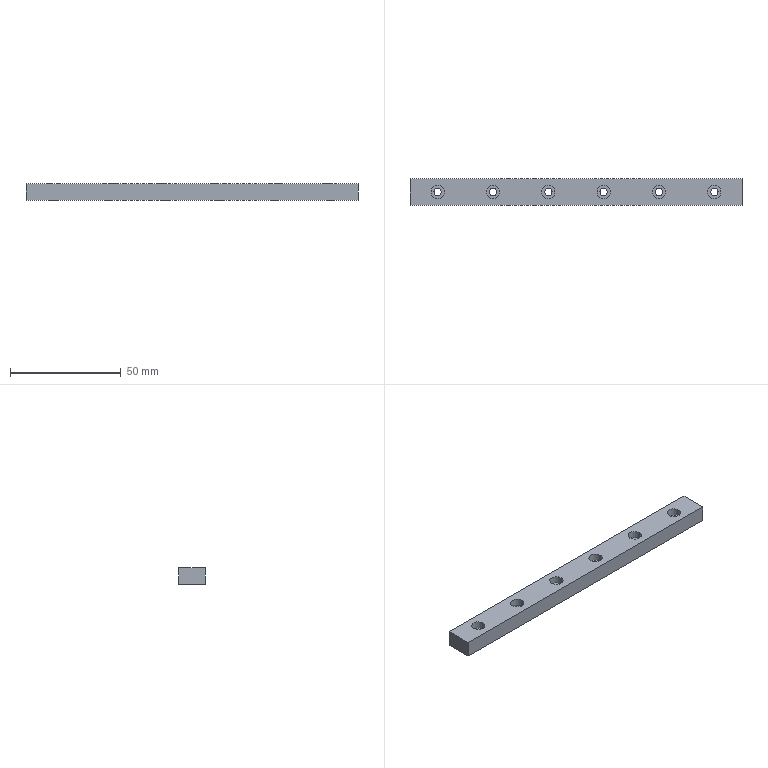Component | SolidWorks | TM12NNA-1-150-NA-Z0-1_TM12NN-150-1 | 1 solid | 36 faces | box 150 x 12 x 7.5 mm | volume 12700 mm3 | cylinder 24 | plane 12 | commonest cylinder face diameters 3.4 x12 6 x12 | material 45
build123d program:
from build123d import *

# Parameters (mm, degrees)
SKETCH1_W                                          = 12
SKETCH1_H                                          = 7.5
BOSS_EXTRUDE1_DEPTH                                = 75
HOLE_SIZE_ACCORDING_TO_TYPE_OF_HEXAGON_D           = 3.4
HOLE_SIZE_ACCORDING_TO_TYPE_OF_HEXAGON_CBORE_D     = 6
HOLE_SIZE_ACCORDING_TO_TYPE_OF_HEXAGON_CBORE_DEPTH = 3.4
LPATTERN1_COUNT                                    = 6
LPATTERN1_PITCH                                    = 25


with BuildPart() as part:
    # Sketch1 → Boss-Extrude1 (new, symmetric)
    with BuildSketch(Plane.XY):
        Rectangle(SKETCH1_W, SKETCH1_H)
    extrude(amount=BOSS_EXTRUDE1_DEPTH, both=True)

    # Hole Size _According to_ Type of Hexagon (through all)
    with Locations(Plane(origin=(0, 3.75, 0), x_dir=(1, 0, 0), z_dir=(0, 1, 0))):
        with Locations((0, -62.5)):
            hole_size_according_to_type_of_hexagon = CounterBoreHole(HOLE_SIZE_ACCORDING_TO_TYPE_OF_HEXAGON_D / 2, HOLE_SIZE_ACCORDING_TO_TYPE_OF_HEXAGON_CBORE_D / 2, HOLE_SIZE_ACCORDING_TO_TYPE_OF_HEXAGON_CBORE_DEPTH)

    # LPattern1: Hole Size _According to_ Type of Hexagon ×6
    with Locations(*[(0, 0, -i * LPATTERN1_PITCH) for i in range(1, LPATTERN1_COUNT)]):
        add(hole_size_according_to_type_of_hexagon, mode=Mode.SUBTRACT)


solid = part.part

# Placed as in the assembly
solid = solid.moved(Location((205, 24, -71.25), (90, -90, 0)))
STEP:
#1=COLOUR_RGB('',0.7922,0.8196,0.9333);
#2=FILL_AREA_STYLE_COLOUR('',#1);
#3=FILL_AREA_STYLE('',(#2));
#4=SURFACE_STYLE_FILL_AREA(#3);
#5=SURFACE_SIDE_STYLE('',(#4));
#6=SURFACE_STYLE_USAGE(.BOTH.,#5);
#7=PRESENTATION_STYLE_ASSIGNMENT((#6));
#8=CARTESIAN_POINT('',(5.543,0.9449,-2.953));
#9=VERTEX_POINT('',#8);
#10=CARTESIAN_POINT('',(5.677,0.9449,-2.953));
#11=VERTEX_POINT('',#10);
#12=CARTESIAN_POINT('',(5.61,0.9449,-2.953));
#13=DIRECTION('',(0.,0.,1.));
#14=DIRECTION('',(1.,0.,0.));
#15=AXIS2_PLACEMENT_3D('',#12,#13,#14);
#16=CIRCLE('',#15,0.06693);
#17=EDGE_CURVE('',#9,#11,#16,.T.);
#18=ORIENTED_EDGE('',*,*,#17,.F.);
#19=CARTESIAN_POINT('',(5.543,0.9449,-2.791));
#20=VERTEX_POINT('',#19);
#21=CARTESIAN_POINT('',(5.543,0.9449,-2.657));
#22=DIRECTION('',(0.,0.,1.));
#23=VECTOR('',#22,39.37);
#24=LINE('',#21,#23);
#25=EDGE_CURVE('',#9,#20,#24,.T.);
#26=ORIENTED_EDGE('',*,*,#25,.T.);
#27=CARTESIAN_POINT('',(5.677,0.9449,-2.791));
#28=VERTEX_POINT('',#27);
#29=CARTESIAN_POINT('',(5.61,0.9449,-2.791));
#30=DIRECTION('',(0.,0.,1.));
#31=DIRECTION('',(1.,0.,0.));
#32=AXIS2_PLACEMENT_3D('',#29,#30,#31);
#33=CIRCLE('',#32,0.06693);
#34=EDGE_CURVE('',#20,#28,#33,.T.);
#35=ORIENTED_EDGE('',*,*,#34,.T.);
#36=CARTESIAN_POINT('',(5.677,0.9449,-2.657));
#37=DIRECTION('',(0.,0.,1.));
#38=VECTOR('',#37,39.37);
#39=LINE('',#36,#38);
#40=EDGE_CURVE('',#11,#28,#39,.T.);
#41=ORIENTED_EDGE('',*,*,#40,.F.);
#42=EDGE_LOOP('',(#18,#26,#35,#41));
#43=FACE_OUTER_BOUND('',#42,.T.);
#44=CARTESIAN_POINT('',(5.61,0.9449,-2.657));
#45=DIRECTION('',(0.,0.,1.));
#46=DIRECTION('',(1.,0.,0.));
#47=AXIS2_PLACEMENT_3D('',#44,#45,#46);
#48=CYLINDRICAL_SURFACE('',#47,0.06693);
#49=ADVANCED_FACE('',(#43),#48,.F.);
#50=CARTESIAN_POINT('',(5.492,0.9449,-2.791));
#51=VERTEX_POINT('',#50);
#52=CARTESIAN_POINT('',(5.728,0.9449,-2.791));
#53=VERTEX_POINT('',#52);
#54=CARTESIAN_POINT('',(5.61,0.9449,-2.791));
#55=DIRECTION('',(0.,0.,1.));
#56=DIRECTION('',(1.,0.,0.));
#57=AXIS2_PLACEMENT_3D('',#54,#55,#56);
#58=CIRCLE('',#57,0.1181);
#59=EDGE_CURVE('',#51,#53,#58,.T.);
#60=ORIENTED_EDGE('',*,*,#59,.F.);
#61=CARTESIAN_POINT('',(5.492,0.9449,-2.657));
#62=VERTEX_POINT('',#61);
#63=CARTESIAN_POINT('',(5.492,0.9449,-2.657));
#64=DIRECTION('',(0.,0.,1.));
#65=VECTOR('',#64,39.37);
#66=LINE('',#63,#65);
#67=EDGE_CURVE('',#51,#62,#66,.T.);
#68=ORIENTED_EDGE('',*,*,#67,.T.);
#69=CARTESIAN_POINT('',(5.728,0.9449,-2.657));
#70=VERTEX_POINT('',#69);
#71=CARTESIAN_POINT('',(5.61,0.9449,-2.657));
#72=DIRECTION('',(0.,0.,1.));
#73=DIRECTION('',(1.,0.,0.));
#74=AXIS2_PLACEMENT_3D('',#71,#72,#73);
#75=CIRCLE('',#74,0.1181);
#76=EDGE_CURVE('',#62,#70,#75,.T.);
#77=ORIENTED_EDGE('',*,*,#76,.T.);
#78=CARTESIAN_POINT('',(5.728,0.9449,-2.657));
#79=DIRECTION('',(0.,0.,1.));
#80=VECTOR('',#79,39.37);
#81=LINE('',#78,#80);
#82=EDGE_CURVE('',#53,#70,#81,.T.);
#83=ORIENTED_EDGE('',*,*,#82,.F.);
#84=EDGE_LOOP('',(#60,#68,#77,#83));
#85=FACE_OUTER_BOUND('',#84,.T.);
#86=CARTESIAN_POINT('',(5.61,0.9449,-2.657));
#87=DIRECTION('',(0.,0.,1.));
#88=DIRECTION('',(1.,0.,0.));
#89=AXIS2_PLACEMENT_3D('',#86,#87,#88);
#90=CYLINDRICAL_SURFACE('',#89,0.1181);
#91=ADVANCED_FACE('',(#85),#90,.F.);
#92=CARTESIAN_POINT('',(6.528,0.9449,-2.953));
#93=VERTEX_POINT('',#92);
#94=CARTESIAN_POINT('',(6.661,0.9449,-2.953));
#95=VERTEX_POINT('',#94);
#96=CARTESIAN_POINT('',(6.594,0.9449,-2.953));
#97=DIRECTION('',(0.,0.,1.));
#98=DIRECTION('',(1.,0.,0.));
#99=AXIS2_PLACEMENT_3D('',#96,#97,#98);
#100=CIRCLE('',#99,0.06693);
#101=EDGE_CURVE('',#93,#95,#100,.T.);
#102=ORIENTED_EDGE('',*,*,#101,.F.);
#103=CARTESIAN_POINT('',(6.528,0.9449,-2.791));
#104=VERTEX_POINT('',#103);
#105=CARTESIAN_POINT('',(6.528,0.9449,-2.657));
#106=DIRECTION('',(0.,0.,1.));
#107=VECTOR('',#106,39.37);
#108=LINE('',#105,#107);
#109=EDGE_CURVE('',#93,#104,#108,.T.);
#110=ORIENTED_EDGE('',*,*,#109,.T.);
#111=CARTESIAN_POINT('',(6.661,0.9449,-2.791));
#112=VERTEX_POINT('',#111);
#113=CARTESIAN_POINT('',(6.594,0.9449,-2.791));
#114=DIRECTION('',(0.,0.,1.));
#115=DIRECTION('',(1.,0.,0.));
#116=AXIS2_PLACEMENT_3D('',#113,#114,#115);
#117=CIRCLE('',#116,0.06693);
#118=EDGE_CURVE('',#104,#112,#117,.T.);
#119=ORIENTED_EDGE('',*,*,#118,.T.);
#120=CARTESIAN_POINT('',(6.661,0.9449,-2.657));
#121=DIRECTION('',(0.,0.,1.));
#122=VECTOR('',#121,39.37);
#123=LINE('',#120,#122);
#124=EDGE_CURVE('',#95,#112,#123,.T.);
#125=ORIENTED_EDGE('',*,*,#124,.F.);
#126=EDGE_LOOP('',(#102,#110,#119,#125));
#127=FACE_OUTER_BOUND('',#126,.T.);
#128=CARTESIAN_POINT('',(6.594,0.9449,-2.657));
#129=DIRECTION('',(0.,0.,1.));
#130=DIRECTION('',(1.,0.,0.));
#131=AXIS2_PLACEMENT_3D('',#128,#129,#130);
#132=CYLINDRICAL_SURFACE('',#131,0.06693);
#133=ADVANCED_FACE('',(#127),#132,.F.);
#134=CARTESIAN_POINT('',(6.476,0.9449,-2.791));
#135=VERTEX_POINT('',#134);
#136=CARTESIAN_POINT('',(6.713,0.9449,-2.791));
#137=VERTEX_POINT('',#136);
#138=CARTESIAN_POINT('',(6.594,0.9449,-2.791));
#139=DIRECTION('',(0.,0.,1.));
#140=DIRECTION('',(1.,0.,0.));
#141=AXIS2_PLACEMENT_3D('',#138,#139,#140);
#142=CIRCLE('',#141,0.1181);
#143=EDGE_CURVE('',#135,#137,#142,.T.);
#144=ORIENTED_EDGE('',*,*,#143,.F.);
#145=CARTESIAN_POINT('',(6.476,0.9449,-2.657));
#146=VERTEX_POINT('',#145);
#147=CARTESIAN_POINT('',(6.476,0.9449,-2.657));
#148=DIRECTION('',(0.,0.,1.));
#149=VECTOR('',#148,39.37);
#150=LINE('',#147,#149);
#151=EDGE_CURVE('',#135,#146,#150,.T.);
#152=ORIENTED_EDGE('',*,*,#151,.T.);
#153=CARTESIAN_POINT('',(6.713,0.9449,-2.657));
#154=VERTEX_POINT('',#153);
#155=CARTESIAN_POINT('',(6.594,0.9449,-2.657));
#156=DIRECTION('',(0.,0.,1.));
#157=DIRECTION('',(1.,0.,0.));
#158=AXIS2_PLACEMENT_3D('',#155,#156,#157);
#159=CIRCLE('',#158,0.1181);
#160=EDGE_CURVE('',#146,#154,#159,.T.);
#161=ORIENTED_EDGE('',*,*,#160,.T.);
#162=CARTESIAN_POINT('',(6.713,0.9449,-2.657));
#163=DIRECTION('',(0.,0.,1.));
#164=VECTOR('',#163,39.37);
#165=LINE('',#162,#164);
#166=EDGE_CURVE('',#137,#154,#165,.T.);
#167=ORIENTED_EDGE('',*,*,#166,.F.);
#168=EDGE_LOOP('',(#144,#152,#161,#167));
#169=FACE_OUTER_BOUND('',#168,.T.);
#170=CARTESIAN_POINT('',(6.594,0.9449,-2.657));
#171=DIRECTION('',(0.,0.,1.));
#172=DIRECTION('',(1.,0.,0.));
#173=AXIS2_PLACEMENT_3D('',#170,#171,#172);
#174=CYLINDRICAL_SURFACE('',#173,0.1181);
#175=ADVANCED_FACE('',(#169),#174,.F.);
#176=CARTESIAN_POINT('',(7.512,0.9449,-2.953));
#177=VERTEX_POINT('',#176);
#178=CARTESIAN_POINT('',(7.646,0.9449,-2.953));
#179=VERTEX_POINT('',#178);
#180=CARTESIAN_POINT('',(7.579,0.9449,-2.953));
#181=DIRECTION('',(0.,0.,1.));
#182=DIRECTION('',(1.,0.,0.));
#183=AXIS2_PLACEMENT_3D('',#180,#181,#182);
#184=CIRCLE('',#183,0.06693);
#185=EDGE_CURVE('',#177,#179,#184,.T.);
#186=ORIENTED_EDGE('',*,*,#185,.F.);
#187=CARTESIAN_POINT('',(7.512,0.9449,-2.791));
#188=VERTEX_POINT('',#187);
#189=CARTESIAN_POINT('',(7.512,0.9449,-2.657));
#190=DIRECTION('',(0.,0.,1.));
#191=VECTOR('',#190,39.37);
#192=LINE('',#189,#191);
#193=EDGE_CURVE('',#177,#188,#192,.T.);
#194=ORIENTED_EDGE('',*,*,#193,.T.);
#195=CARTESIAN_POINT('',(7.646,0.9449,-2.791));
#196=VERTEX_POINT('',#195);
#197=CARTESIAN_POINT('',(7.579,0.9449,-2.791));
#198=DIRECTION('',(0.,0.,1.));
#199=DIRECTION('',(1.,0.,0.));
#200=AXIS2_PLACEMENT_3D('',#197,#198,#199);
#201=CIRCLE('',#200,0.06693);
#202=EDGE_CURVE('',#188,#196,#201,.T.);
#203=ORIENTED_EDGE('',*,*,#202,.T.);
#204=CARTESIAN_POINT('',(7.646,0.9449,-2.657));
#205=DIRECTION('',(0.,0.,1.));
#206=VECTOR('',#205,39.37);
#207=LINE('',#204,#206);
#208=EDGE_CURVE('',#179,#196,#207,.T.);
#209=ORIENTED_EDGE('',*,*,#208,.F.);
#210=EDGE_LOOP('',(#186,#194,#203,#209));
#211=FACE_OUTER_BOUND('',#210,.T.);
#212=CARTESIAN_POINT('',(7.579,0.9449,-2.657));
#213=DIRECTION('',(0.,0.,1.));
#214=DIRECTION('',(1.,0.,0.));
#215=AXIS2_PLACEMENT_3D('',#212,#213,#214);
#216=CYLINDRICAL_SURFACE('',#215,0.06693);
#217=ADVANCED_FACE('',(#211),#216,.F.);
#218=CARTESIAN_POINT('',(7.461,0.9449,-2.791));
#219=VERTEX_POINT('',#218);
#220=CARTESIAN_POINT('',(7.697,0.9449,-2.791));
#221=VERTEX_POINT('',#220);
#222=CARTESIAN_POINT('',(7.579,0.9449,-2.791));
#223=DIRECTION('',(0.,0.,1.));
#224=DIRECTION('',(1.,0.,0.));
#225=AXIS2_PLACEMENT_3D('',#222,#223,#224);
#226=CIRCLE('',#225,0.1181);
#227=EDGE_CURVE('',#219,#221,#226,.T.);
#228=ORIENTED_EDGE('',*,*,#227,.F.);
#229=CARTESIAN_POINT('',(7.461,0.9449,-2.657));
#230=VERTEX_POINT('',#229);
#231=CARTESIAN_POINT('',(7.461,0.9449,-2.657));
#232=DIRECTION('',(0.,0.,1.));
#233=VECTOR('',#232,39.37);
#234=LINE('',#231,#233);
#235=EDGE_CURVE('',#219,#230,#234,.T.);
#236=ORIENTED_EDGE('',*,*,#235,.T.);
#237=CARTESIAN_POINT('',(7.697,0.9449,-2.657));
#238=VERTEX_POINT('',#237);
#239=CARTESIAN_POINT('',(7.579,0.9449,-2.657));
#240=DIRECTION('',(0.,0.,1.));
#241=DIRECTION('',(1.,0.,0.));
#242=AXIS2_PLACEMENT_3D('',#239,#240,#241);
#243=CIRCLE('',#242,0.1181);
#244=EDGE_CURVE('',#230,#238,#243,.T.);
#245=ORIENTED_EDGE('',*,*,#244,.T.);
#246=CARTESIAN_POINT('',(7.697,0.9449,-2.657));
#247=DIRECTION('',(0.,0.,1.));
#248=VECTOR('',#247,39.37);
#249=LINE('',#246,#248);
#250=EDGE_CURVE('',#221,#238,#249,.T.);
#251=ORIENTED_EDGE('',*,*,#250,.F.);
#252=EDGE_LOOP('',(#228,#236,#245,#251));
#253=FACE_OUTER_BOUND('',#252,.T.);
#254=CARTESIAN_POINT('',(7.579,0.9449,-2.657));
#255=DIRECTION('',(0.,0.,1.));
#256=DIRECTION('',(1.,0.,0.));
#257=AXIS2_PLACEMENT_3D('',#254,#255,#256);
#258=CYLINDRICAL_SURFACE('',#257,0.1181);
#259=ADVANCED_FACE('',(#253),#258,.F.);
#260=CARTESIAN_POINT('',(8.496,0.9449,-2.953));
#261=VERTEX_POINT('',#260);
#262=CARTESIAN_POINT('',(8.63,0.9449,-2.953));
#263=VERTEX_POINT('',#262);
#264=CARTESIAN_POINT('',(8.563,0.9449,-2.953));
#265=DIRECTION('',(0.,0.,1.));
#266=DIRECTION('',(1.,0.,0.));
#267=AXIS2_PLACEMENT_3D('',#264,#265,#266);
#268=CIRCLE('',#267,0.06693);
#269=EDGE_CURVE('',#261,#263,#268,.T.);
#270=ORIENTED_EDGE('',*,*,#269,.F.);
#271=CARTESIAN_POINT('',(8.496,0.9449,-2.791));
#272=VERTEX_POINT('',#271);
#273=CARTESIAN_POINT('',(8.496,0.9449,-2.657));
#274=DIRECTION('',(0.,0.,1.));
#275=VECTOR('',#274,39.37);
#276=LINE('',#273,#275);
#277=EDGE_CURVE('',#261,#272,#276,.T.);
#278=ORIENTED_EDGE('',*,*,#277,.T.);
#279=CARTESIAN_POINT('',(8.63,0.9449,-2.791));
#280=VERTEX_POINT('',#279);
#281=CARTESIAN_POINT('',(8.563,0.9449,-2.791));
#282=DIRECTION('',(0.,0.,1.));
#283=DIRECTION('',(1.,0.,0.));
#284=AXIS2_PLACEMENT_3D('',#281,#282,#283);
#285=CIRCLE('',#284,0.06693);
#286=EDGE_CURVE('',#272,#280,#285,.T.);
#287=ORIENTED_EDGE('',*,*,#286,.T.);
#288=CARTESIAN_POINT('',(8.63,0.9449,-2.657));
#289=DIRECTION('',(0.,0.,1.));
#290=VECTOR('',#289,39.37);
#291=LINE('',#288,#290);
#292=EDGE_CURVE('',#263,#280,#291,.T.);
#293=ORIENTED_EDGE('',*,*,#292,.F.);
#294=EDGE_LOOP('',(#270,#278,#287,#293));
#295=FACE_OUTER_BOUND('',#294,.T.);
#296=CARTESIAN_POINT('',(8.563,0.9449,-2.657));
#297=DIRECTION('',(0.,0.,1.));
#298=DIRECTION('',(1.,0.,0.));
#299=AXIS2_PLACEMENT_3D('',#296,#297,#298);
#300=CYLINDRICAL_SURFACE('',#299,0.06693);
#301=ADVANCED_FACE('',(#295),#300,.F.);
#302=CARTESIAN_POINT('',(8.445,0.9449,-2.791));
#303=VERTEX_POINT('',#302);
#304=CARTESIAN_POINT('',(8.681,0.9449,-2.791));
#305=VERTEX_POINT('',#304);
#306=CARTESIAN_POINT('',(8.563,0.9449,-2.791));
#307=DIRECTION('',(0.,0.,1.));
#308=DIRECTION('',(1.,0.,0.));
#309=AXIS2_PLACEMENT_3D('',#306,#307,#308);
#310=CIRCLE('',#309,0.1181);
#311=EDGE_CURVE('',#303,#305,#310,.T.);
#312=ORIENTED_EDGE('',*,*,#311,.F.);
#313=CARTESIAN_POINT('',(8.445,0.9449,-2.657));
#314=VERTEX_POINT('',#313);
#315=CARTESIAN_POINT('',(8.445,0.9449,-2.657));
#316=DIRECTION('',(0.,0.,1.));
#317=VECTOR('',#316,39.37);
#318=LINE('',#315,#317);
#319=EDGE_CURVE('',#303,#314,#318,.T.);
#320=ORIENTED_EDGE('',*,*,#319,.T.);
#321=CARTESIAN_POINT('',(8.681,0.9449,-2.657));
#322=VERTEX_POINT('',#321);
#323=CARTESIAN_POINT('',(8.563,0.9449,-2.657));
#324=DIRECTION('',(0.,0.,1.));
#325=DIRECTION('',(1.,0.,0.));
#326=AXIS2_PLACEMENT_3D('',#323,#324,#325);
#327=CIRCLE('',#326,0.1181);
#328=EDGE_CURVE('',#314,#322,#327,.T.);
#329=ORIENTED_EDGE('',*,*,#328,.T.);
#330=CARTESIAN_POINT('',(8.681,0.9449,-2.657));
#331=DIRECTION('',(0.,0.,1.));
#332=VECTOR('',#331,39.37);
#333=LINE('',#330,#332);
#334=EDGE_CURVE('',#305,#322,#333,.T.);
#335=ORIENTED_EDGE('',*,*,#334,.F.);
#336=EDGE_LOOP('',(#312,#320,#329,#335));
#337=FACE_OUTER_BOUND('',#336,.T.);
#338=CARTESIAN_POINT('',(8.563,0.9449,-2.657));
#339=DIRECTION('',(0.,0.,1.));
#340=DIRECTION('',(1.,0.,0.));
#341=AXIS2_PLACEMENT_3D('',#338,#339,#340);
#342=CYLINDRICAL_SURFACE('',#341,0.1181);
#343=ADVANCED_FACE('',(#337),#342,.F.);
#344=CARTESIAN_POINT('',(9.429,0.9449,-2.791));
#345=VERTEX_POINT('',#344);
#346=CARTESIAN_POINT('',(9.665,0.9449,-2.791));
#347=VERTEX_POINT('',#346);
#348=CARTESIAN_POINT('',(9.547,0.9449,-2.791));
#349=DIRECTION('',(0.,0.,1.));
#350=DIRECTION('',(1.,0.,0.));
#351=AXIS2_PLACEMENT_3D('',#348,#349,#350);
#352=CIRCLE('',#351,0.1181);
#353=EDGE_CURVE('',#345,#347,#352,.T.);
#354=ORIENTED_EDGE('',*,*,#353,.F.);
#355=CARTESIAN_POINT('',(9.429,0.9449,-2.657));
#356=VERTEX_POINT('',#355);
#357=CARTESIAN_POINT('',(9.429,0.9449,-2.657));
#358=DIRECTION('',(0.,0.,1.));
#359=VECTOR('',#358,39.37);
#360=LINE('',#357,#359);
#361=EDGE_CURVE('',#345,#356,#360,.T.);
#362=ORIENTED_EDGE('',*,*,#361,.T.);
#363=CARTESIAN_POINT('',(9.665,0.9449,-2.657));
#364=VERTEX_POINT('',#363);
#365=CARTESIAN_POINT('',(9.547,0.9449,-2.657));
#366=DIRECTION('',(0.,0.,1.));
#367=DIRECTION('',(1.,0.,0.));
#368=AXIS2_PLACEMENT_3D('',#365,#366,#367);
#369=CIRCLE('',#368,0.1181);
#370=EDGE_CURVE('',#356,#364,#369,.T.);
#371=ORIENTED_EDGE('',*,*,#370,.T.);
#372=CARTESIAN_POINT('',(9.665,0.9449,-2.657));
#373=DIRECTION('',(0.,0.,1.));
#374=VECTOR('',#373,39.37);
#375=LINE('',#372,#374);
#376=EDGE_CURVE('',#347,#364,#375,.T.);
#377=ORIENTED_EDGE('',*,*,#376,.F.);
#378=EDGE_LOOP('',(#354,#362,#371,#377));
#379=FACE_OUTER_BOUND('',#378,.T.);
#380=CARTESIAN_POINT('',(9.547,0.9449,-2.657));
#381=DIRECTION('',(0.,0.,1.));
#382=DIRECTION('',(1.,0.,0.));
#383=AXIS2_PLACEMENT_3D('',#380,#381,#382);
#384=CYLINDRICAL_SURFACE('',#383,0.1181);
#385=ADVANCED_FACE('',(#379),#384,.F.);
#386=CARTESIAN_POINT('',(9.48,0.9449,-2.953));
#387=VERTEX_POINT('',#386);
#388=CARTESIAN_POINT('',(9.614,0.9449,-2.953));
#389=VERTEX_POINT('',#388);
#390=CARTESIAN_POINT('',(9.547,0.9449,-2.953));
#391=DIRECTION('',(0.,0.,1.));
#392=DIRECTION('',(1.,0.,0.));
#393=AXIS2_PLACEMENT_3D('',#390,#391,#392);
#394=CIRCLE('',#393,0.06693);
#395=EDGE_CURVE('',#387,#389,#394,.T.);
#396=ORIENTED_EDGE('',*,*,#395,.F.);
#397=CARTESIAN_POINT('',(9.48,0.9449,-2.791));
#398=VERTEX_POINT('',#397);
#399=CARTESIAN_POINT('',(9.48,0.9449,-2.657));
#400=DIRECTION('',(0.,0.,1.));
#401=VECTOR('',#400,39.37);
#402=LINE('',#399,#401);
#403=EDGE_CURVE('',#387,#398,#402,.T.);
#404=ORIENTED_EDGE('',*,*,#403,.T.);
#405=CARTESIAN_POINT('',(9.614,0.9449,-2.791));
#406=VERTEX_POINT('',#405);
#407=CARTESIAN_POINT('',(9.547,0.9449,-2.791));
#408=DIRECTION('',(0.,0.,1.));
#409=DIRECTION('',(1.,0.,0.));
#410=AXIS2_PLACEMENT_3D('',#407,#408,#409);
#411=CIRCLE('',#410,0.06693);
#412=EDGE_CURVE('',#398,#406,#411,.T.);
#413=ORIENTED_EDGE('',*,*,#412,.T.);
#414=CARTESIAN_POINT('',(9.614,0.9449,-2.657));
#415=DIRECTION('',(0.,0.,1.));
#416=VECTOR('',#415,39.37);
#417=LINE('',#414,#416);
#418=EDGE_CURVE('',#389,#406,#417,.T.);
#419=ORIENTED_EDGE('',*,*,#418,.F.);
#420=EDGE_LOOP('',(#396,#404,#413,#419));
#421=FACE_OUTER_BOUND('',#420,.T.);
#422=CARTESIAN_POINT('',(9.547,0.9449,-2.657));
#423=DIRECTION('',(0.,0.,1.));
#424=DIRECTION('',(1.,0.,0.));
#425=AXIS2_PLACEMENT_3D('',#422,#423,#424);
#426=CYLINDRICAL_SURFACE('',#425,0.06693);
#427=ADVANCED_FACE('',(#421),#426,.F.);
#428=CARTESIAN_POINT('',(10.413,0.9449,-2.791));
#429=VERTEX_POINT('',#428);
#430=CARTESIAN_POINT('',(10.65,0.9449,-2.791));
#431=VERTEX_POINT('',#430);
#432=CARTESIAN_POINT('',(10.531,0.9449,-2.791));
#433=DIRECTION('',(0.,0.,1.));
#434=DIRECTION('',(1.,0.,0.));
#435=AXIS2_PLACEMENT_3D('',#432,#433,#434);
#436=CIRCLE('',#435,0.1181);
#437=EDGE_CURVE('',#429,#431,#436,.T.);
#438=ORIENTED_EDGE('',*,*,#437,.F.);
#439=CARTESIAN_POINT('',(10.413,0.9449,-2.657));
#440=VERTEX_POINT('',#439);
#441=CARTESIAN_POINT('',(10.413,0.9449,-2.657));
#442=DIRECTION('',(0.,0.,1.));
#443=VECTOR('',#442,39.37);
#444=LINE('',#441,#443);
#445=EDGE_CURVE('',#429,#440,#444,.T.);
#446=ORIENTED_EDGE('',*,*,#445,.T.);
#447=CARTESIAN_POINT('',(10.65,0.9449,-2.657));
#448=VERTEX_POINT('',#447);
#449=CARTESIAN_POINT('',(10.531,0.9449,-2.657));
#450=DIRECTION('',(0.,0.,1.));
#451=DIRECTION('',(1.,0.,0.));
#452=AXIS2_PLACEMENT_3D('',#449,#450,#451);
#453=CIRCLE('',#452,0.1181);
#454=EDGE_CURVE('',#440,#448,#453,.T.);
#455=ORIENTED_EDGE('',*,*,#454,.T.);
#456=CARTESIAN_POINT('',(10.65,0.9449,-2.657));
#457=DIRECTION('',(0.,0.,1.));
#458=VECTOR('',#457,39.37);
#459=LINE('',#456,#458);
#460=EDGE_CURVE('',#431,#448,#459,.T.);
#461=ORIENTED_EDGE('',*,*,#460,.F.);
#462=EDGE_LOOP('',(#438,#446,#455,#461));
#463=FACE_OUTER_BOUND('',#462,.T.);
#464=CARTESIAN_POINT('',(10.531,0.9449,-2.657));
#465=DIRECTION('',(0.,0.,1.));
#466=DIRECTION('',(1.,0.,0.));
#467=AXIS2_PLACEMENT_3D('',#464,#465,#466);
#468=CYLINDRICAL_SURFACE('',#467,0.1181);
#469=ADVANCED_FACE('',(#463),#468,.F.);
#470=CARTESIAN_POINT('',(10.465,0.9449,-2.953));
#471=VERTEX_POINT('',#470);
#472=CARTESIAN_POINT('',(10.598,0.9449,-2.953));
#473=VERTEX_POINT('',#472);
#474=CARTESIAN_POINT('',(10.531,0.9449,-2.953));
#475=DIRECTION('',(0.,0.,1.));
#476=DIRECTION('',(1.,0.,0.));
#477=AXIS2_PLACEMENT_3D('',#474,#475,#476);
#478=CIRCLE('',#477,0.06693);
#479=EDGE_CURVE('',#471,#473,#478,.T.);
#480=ORIENTED_EDGE('',*,*,#479,.F.);
#481=CARTESIAN_POINT('',(10.465,0.9449,-2.791));
#482=VERTEX_POINT('',#481);
#483=CARTESIAN_POINT('',(10.465,0.9449,-2.657));
#484=DIRECTION('',(0.,0.,1.));
#485=VECTOR('',#484,39.37);
#486=LINE('',#483,#485);
#487=EDGE_CURVE('',#471,#482,#486,.T.);
#488=ORIENTED_EDGE('',*,*,#487,.T.);
#489=CARTESIAN_POINT('',(10.598,0.9449,-2.791));
#490=VERTEX_POINT('',#489);
#491=CARTESIAN_POINT('',(10.531,0.9449,-2.791));
#492=DIRECTION('',(0.,0.,1.));
#493=DIRECTION('',(1.,0.,0.));
#494=AXIS2_PLACEMENT_3D('',#491,#492,#493);
#495=CIRCLE('',#494,0.06693);
#496=EDGE_CURVE('',#482,#490,#495,.T.);
#497=ORIENTED_EDGE('',*,*,#496,.T.);
#498=CARTESIAN_POINT('',(10.598,0.9449,-2.657));
#499=DIRECTION('',(0.,0.,1.));
#500=VECTOR('',#499,39.37);
#501=LINE('',#498,#500);
#502=EDGE_CURVE('',#473,#490,#501,.T.);
#503=ORIENTED_EDGE('',*,*,#502,.F.);
#504=EDGE_LOOP('',(#480,#488,#497,#503));
#505=FACE_OUTER_BOUND('',#504,.T.);
#506=CARTESIAN_POINT('',(10.531,0.9449,-2.657));
#507=DIRECTION('',(0.,0.,1.));
#508=DIRECTION('',(1.,0.,0.));
#509=AXIS2_PLACEMENT_3D('',#506,#507,#508);
#510=CYLINDRICAL_SURFACE('',#509,0.06693);
#511=ADVANCED_FACE('',(#505),#510,.F.);
#512=CARTESIAN_POINT('',(5.118,1.181,-2.953));
#513=VERTEX_POINT('',#512);
#514=CARTESIAN_POINT('',(5.118,1.181,-2.657));
#515=VERTEX_POINT('',#514);
#516=CARTESIAN_POINT('',(5.118,1.181,-2.953));
#517=DIRECTION('',(0.,0.,1.));
#518=VECTOR('',#517,39.37);
#519=LINE('',#516,#518);
#520=EDGE_CURVE('',#513,#515,#519,.T.);
#521=ORIENTED_EDGE('',*,*,#520,.T.);
#522=CARTESIAN_POINT('',(11.024,1.181,-2.657));
#523=VERTEX_POINT('',#522);
#524=CARTESIAN_POINT('',(11.024,1.181,-2.657));
#525=DIRECTION('',(-1.,0.,0.));
#526=VECTOR('',#525,39.37);
#527=LINE('',#524,#526);
#528=EDGE_CURVE('',#523,#515,#527,.T.);
#529=ORIENTED_EDGE('',*,*,#528,.F.);
#530=CARTESIAN_POINT('',(11.024,1.181,-2.953));
#531=VERTEX_POINT('',#530);
#532=CARTESIAN_POINT('',(11.024,1.181,-2.953));
#533=DIRECTION('',(0.,0.,1.));
#534=VECTOR('',#533,39.37);
#535=LINE('',#532,#534);
#536=EDGE_CURVE('',#531,#523,#535,.T.);
#537=ORIENTED_EDGE('',*,*,#536,.F.);
#538=CARTESIAN_POINT('',(11.024,1.181,-2.953));
#539=DIRECTION('',(-1.,0.,0.));
#540=VECTOR('',#539,39.37);
#541=LINE('',#538,#540);
#542=EDGE_CURVE('',#531,#513,#541,.T.);
#543=ORIENTED_EDGE('',*,*,#542,.T.);
#544=EDGE_LOOP('',(#521,#529,#537,#543));
#545=FACE_OUTER_BOUND('',#544,.T.);
#546=CARTESIAN_POINT('',(11.024,1.181,-2.953));
#547=DIRECTION('',(0.,-1.,0.));
#548=DIRECTION('',(1.,0.,0.));
#549=AXIS2_PLACEMENT_3D('',#546,#547,#548);
#550=PLANE('',#549);
#551=ADVANCED_FACE('',(#545),#550,.F.);
#552=CARTESIAN_POINT('',(9.547,0.9449,-2.657));
#553=DIRECTION('',(0.,0.,1.));
#554=DIRECTION('',(1.,0.,0.));
#555=AXIS2_PLACEMENT_3D('',#552,#553,#554);
#556=CIRCLE('',#555,0.1181);
#557=EDGE_CURVE('',#364,#356,#556,.T.);
#558=ORIENTED_EDGE('',*,*,#557,.F.);
#559=ORIENTED_EDGE('',*,*,#370,.F.);
#560=EDGE_LOOP('',(#558,#559));
#561=FACE_BOUND('',#560,.T.);
#562=CARTESIAN_POINT('',(10.531,0.9449,-2.657));
#563=DIRECTION('',(0.,0.,1.));
#564=DIRECTION('',(1.,0.,0.));
#565=AXIS2_PLACEMENT_3D('',#562,#563,#564);
#566=CIRCLE('',#565,0.1181);
#567=EDGE_CURVE('',#448,#440,#566,.T.);
#568=ORIENTED_EDGE('',*,*,#567,.F.);
#569=ORIENTED_EDGE('',*,*,#454,.F.);
#570=EDGE_LOOP('',(#568,#569));
#571=FACE_BOUND('',#570,.T.);
#572=CARTESIAN_POINT('',(5.118,0.7087,-2.657));
#573=VERTEX_POINT('',#572);
#574=CARTESIAN_POINT('',(5.118,0.7087,-2.657));
#575=DIRECTION('',(0.,-1.,0.));
#576=VECTOR('',#575,39.37);
#577=LINE('',#574,#576);
#578=EDGE_CURVE('',#515,#573,#577,.T.);
#579=ORIENTED_EDGE('',*,*,#578,.T.);
#580=CARTESIAN_POINT('',(11.024,0.7087,-2.657));
#581=VERTEX_POINT('',#580);
#582=CARTESIAN_POINT('',(11.024,0.7087,-2.657));
#583=DIRECTION('',(-1.,0.,0.));
#584=VECTOR('',#583,39.37);
#585=LINE('',#582,#584);
#586=EDGE_CURVE('',#581,#573,#585,.T.);
#587=ORIENTED_EDGE('',*,*,#586,.F.);
#588=CARTESIAN_POINT('',(11.024,0.7087,-2.657));
#589=DIRECTION('',(0.,-1.,0.));
#590=VECTOR('',#589,39.37);
#591=LINE('',#588,#590);
#592=EDGE_CURVE('',#523,#581,#591,.T.);
#593=ORIENTED_EDGE('',*,*,#592,.F.);
#594=ORIENTED_EDGE('',*,*,#528,.T.);
#595=EDGE_LOOP('',(#579,#587,#593,#594));
#596=FACE_OUTER_BOUND('',#595,.T.);
#597=CARTESIAN_POINT('',(8.563,0.9449,-2.657));
#598=DIRECTION('',(0.,0.,1.));
#599=DIRECTION('',(1.,0.,0.));
#600=AXIS2_PLACEMENT_3D('',#597,#598,#599);
#601=CIRCLE('',#600,0.1181);
#602=EDGE_CURVE('',#322,#314,#601,.T.);
#603=ORIENTED_EDGE('',*,*,#602,.F.);
#604=ORIENTED_EDGE('',*,*,#328,.F.);
#605=EDGE_LOOP('',(#603,#604));
#606=FACE_BOUND('',#605,.T.);
#607=CARTESIAN_POINT('',(7.579,0.9449,-2.657));
#608=DIRECTION('',(0.,0.,1.));
#609=DIRECTION('',(1.,0.,0.));
#610=AXIS2_PLACEMENT_3D('',#607,#608,#609);
#611=CIRCLE('',#610,0.1181);
#612=EDGE_CURVE('',#238,#230,#611,.T.);
#613=ORIENTED_EDGE('',*,*,#612,.F.);
#614=ORIENTED_EDGE('',*,*,#244,.F.);
#615=EDGE_LOOP('',(#613,#614));
#616=FACE_BOUND('',#615,.T.);
#617=CARTESIAN_POINT('',(6.594,0.9449,-2.657));
#618=DIRECTION('',(0.,0.,1.));
#619=DIRECTION('',(1.,0.,0.));
#620=AXIS2_PLACEMENT_3D('',#617,#618,#619);
#621=CIRCLE('',#620,0.1181);
#622=EDGE_CURVE('',#154,#146,#621,.T.);
#623=ORIENTED_EDGE('',*,*,#622,.F.);
#624=ORIENTED_EDGE('',*,*,#160,.F.);
#625=EDGE_LOOP('',(#623,#624));
#626=FACE_BOUND('',#625,.T.);
#627=CARTESIAN_POINT('',(5.61,0.9449,-2.657));
#628=DIRECTION('',(0.,0.,1.));
#629=DIRECTION('',(1.,0.,0.));
#630=AXIS2_PLACEMENT_3D('',#627,#628,#629);
#631=CIRCLE('',#630,0.1181);
#632=EDGE_CURVE('',#70,#62,#631,.T.);
#633=ORIENTED_EDGE('',*,*,#632,.F.);
#634=ORIENTED_EDGE('',*,*,#76,.F.);
#635=EDGE_LOOP('',(#633,#634));
#636=FACE_BOUND('',#635,.T.);
#637=CARTESIAN_POINT('',(11.024,0.7087,-2.657));
#638=DIRECTION('',(0.,0.,-1.));
#639=DIRECTION('',(-1.,0.,0.));
#640=AXIS2_PLACEMENT_3D('',#637,#638,#639);
#641=PLANE('',#640);
#642=ADVANCED_FACE('',(#561,#571,#596,#606,#616,#626,#636),#641,.F.);
#643=CARTESIAN_POINT('',(5.118,0.7087,-2.953));
#644=VERTEX_POINT('',#643);
#645=CARTESIAN_POINT('',(5.118,0.7087,-2.953));
#646=DIRECTION('',(0.,0.,-1.));
#647=VECTOR('',#646,39.37);
#648=LINE('',#645,#647);
#649=EDGE_CURVE('',#573,#644,#648,.T.);
#650=ORIENTED_EDGE('',*,*,#649,.T.);
#651=CARTESIAN_POINT('',(11.024,0.7087,-2.953));
#652=VERTEX_POINT('',#651);
#653=CARTESIAN_POINT('',(11.024,0.7087,-2.953));
#654=DIRECTION('',(-1.,0.,0.));
#655=VECTOR('',#654,39.37);
#656=LINE('',#653,#655);
#657=EDGE_CURVE('',#652,#644,#656,.T.);
#658=ORIENTED_EDGE('',*,*,#657,.F.);
#659=CARTESIAN_POINT('',(11.024,0.7087,-2.953));
#660=DIRECTION('',(0.,0.,-1.));
#661=VECTOR('',#660,39.37);
#662=LINE('',#659,#661);
#663=EDGE_CURVE('',#581,#652,#662,.T.);
#664=ORIENTED_EDGE('',*,*,#663,.F.);
#665=ORIENTED_EDGE('',*,*,#586,.T.);
#666=EDGE_LOOP('',(#650,#658,#664,#665));
#667=FACE_OUTER_BOUND('',#666,.T.);
#668=CARTESIAN_POINT('',(11.024,0.7087,-2.953));
#669=DIRECTION('',(0.,1.,0.));
#670=DIRECTION('',(-1.,0.,0.));
#671=AXIS2_PLACEMENT_3D('',#668,#669,#670);
#672=PLANE('',#671);
#673=ADVANCED_FACE('',(#667),#672,.F.);
#674=CARTESIAN_POINT('',(9.547,0.9449,-2.953));
#675=DIRECTION('',(0.,0.,1.));
#676=DIRECTION('',(1.,0.,0.));
#677=AXIS2_PLACEMENT_3D('',#674,#675,#676);
#678=CIRCLE('',#677,0.06693);
#679=EDGE_CURVE('',#389,#387,#678,.T.);
#680=ORIENTED_EDGE('',*,*,#679,.T.);
#681=ORIENTED_EDGE('',*,*,#395,.T.);
#682=EDGE_LOOP('',(#680,#681));
#683=FACE_BOUND('',#682,.T.);
#684=CARTESIAN_POINT('',(10.531,0.9449,-2.953));
#685=DIRECTION('',(0.,0.,1.));
#686=DIRECTION('',(1.,0.,0.));
#687=AXIS2_PLACEMENT_3D('',#684,#685,#686);
#688=CIRCLE('',#687,0.06693);
#689=EDGE_CURVE('',#473,#471,#688,.T.);
#690=ORIENTED_EDGE('',*,*,#689,.T.);
#691=ORIENTED_EDGE('',*,*,#479,.T.);
#692=EDGE_LOOP('',(#690,#691));
#693=FACE_BOUND('',#692,.T.);
#694=CARTESIAN_POINT('',(5.118,0.7087,-2.953));
#695=DIRECTION('',(0.,1.,0.));
#696=VECTOR('',#695,39.37);
#697=LINE('',#694,#696);
#698=EDGE_CURVE('',#644,#513,#697,.T.);
#699=ORIENTED_EDGE('',*,*,#698,.T.);
#700=ORIENTED_EDGE('',*,*,#542,.F.);
#701=CARTESIAN_POINT('',(11.024,0.7087,-2.953));
#702=DIRECTION('',(0.,1.,0.));
#703=VECTOR('',#702,39.37);
#704=LINE('',#701,#703);
#705=EDGE_CURVE('',#652,#531,#704,.T.);
#706=ORIENTED_EDGE('',*,*,#705,.F.);
#707=ORIENTED_EDGE('',*,*,#657,.T.);
#708=EDGE_LOOP('',(#699,#700,#706,#707));
#709=FACE_OUTER_BOUND('',#708,.T.);
#710=CARTESIAN_POINT('',(8.563,0.9449,-2.953));
#711=DIRECTION('',(0.,0.,1.));
#712=DIRECTION('',(1.,0.,0.));
#713=AXIS2_PLACEMENT_3D('',#710,#711,#712);
#714=CIRCLE('',#713,0.06693);
#715=EDGE_CURVE('',#263,#261,#714,.T.);
#716=ORIENTED_EDGE('',*,*,#715,.T.);
#717=ORIENTED_EDGE('',*,*,#269,.T.);
#718=EDGE_LOOP('',(#716,#717));
#719=FACE_BOUND('',#718,.T.);
#720=CARTESIAN_POINT('',(7.579,0.9449,-2.953));
#721=DIRECTION('',(0.,0.,1.));
#722=DIRECTION('',(1.,0.,0.));
#723=AXIS2_PLACEMENT_3D('',#720,#721,#722);
#724=CIRCLE('',#723,0.06693);
#725=EDGE_CURVE('',#179,#177,#724,.T.);
#726=ORIENTED_EDGE('',*,*,#725,.T.);
#727=ORIENTED_EDGE('',*,*,#185,.T.);
#728=EDGE_LOOP('',(#726,#727));
#729=FACE_BOUND('',#728,.T.);
#730=CARTESIAN_POINT('',(6.594,0.9449,-2.953));
#731=DIRECTION('',(0.,0.,1.));
#732=DIRECTION('',(1.,0.,0.));
#733=AXIS2_PLACEMENT_3D('',#730,#731,#732);
#734=CIRCLE('',#733,0.06693);
#735=EDGE_CURVE('',#95,#93,#734,.T.);
#736=ORIENTED_EDGE('',*,*,#735,.T.);
#737=ORIENTED_EDGE('',*,*,#101,.T.);
#738=EDGE_LOOP('',(#736,#737));
#739=FACE_BOUND('',#738,.T.);
#740=CARTESIAN_POINT('',(5.61,0.9449,-2.953));
#741=DIRECTION('',(0.,0.,1.));
#742=DIRECTION('',(1.,0.,0.));
#743=AXIS2_PLACEMENT_3D('',#740,#741,#742);
#744=CIRCLE('',#743,0.06693);
#745=EDGE_CURVE('',#11,#9,#744,.T.);
#746=ORIENTED_EDGE('',*,*,#745,.T.);
#747=ORIENTED_EDGE('',*,*,#17,.T.);
#748=EDGE_LOOP('',(#746,#747));
#749=FACE_BOUND('',#748,.T.);
#750=CARTESIAN_POINT('',(11.024,0.7087,-2.953));
#751=DIRECTION('',(0.,0.,1.));
#752=DIRECTION('',(1.,0.,0.));
#753=AXIS2_PLACEMENT_3D('',#750,#751,#752);
#754=PLANE('',#753);
#755=ADVANCED_FACE('',(#683,#693,#709,#719,#729,#739,#749),#754,.F.);
#756=ORIENTED_EDGE('',*,*,#536,.T.);
#757=ORIENTED_EDGE('',*,*,#592,.T.);
#758=ORIENTED_EDGE('',*,*,#663,.T.);
#759=ORIENTED_EDGE('',*,*,#705,.T.);
#760=EDGE_LOOP('',(#756,#757,#758,#759));
#761=FACE_OUTER_BOUND('',#760,.T.);
#762=CARTESIAN_POINT('',(11.024,0.9449,-2.805));
#763=DIRECTION('',(-1.,0.,0.));
#764=DIRECTION('',(0.,-1.,0.));
#765=AXIS2_PLACEMENT_3D('',#762,#763,#764);
#766=PLANE('',#765);
#767=ADVANCED_FACE('',(#761),#766,.F.);
#768=ORIENTED_EDGE('',*,*,#520,.F.);
#769=ORIENTED_EDGE('',*,*,#698,.F.);
#770=ORIENTED_EDGE('',*,*,#649,.F.);
#771=ORIENTED_EDGE('',*,*,#578,.F.);
#772=EDGE_LOOP('',(#768,#769,#770,#771));
#773=FACE_OUTER_BOUND('',#772,.T.);
#774=CARTESIAN_POINT('',(5.118,0.9449,-2.805));
#775=DIRECTION('',(-1.,0.,0.));
#776=DIRECTION('',(0.,-1.,0.));
#777=AXIS2_PLACEMENT_3D('',#774,#775,#776);
#778=PLANE('',#777);
#779=ADVANCED_FACE('',(#773),#778,.T.);
#780=ORIENTED_EDGE('',*,*,#487,.F.);
#781=ORIENTED_EDGE('',*,*,#689,.F.);
#782=ORIENTED_EDGE('',*,*,#502,.T.);
#783=CARTESIAN_POINT('',(10.531,0.9449,-2.791));
#784=DIRECTION('',(0.,0.,1.));
#785=DIRECTION('',(1.,0.,0.));
#786=AXIS2_PLACEMENT_3D('',#783,#784,#785);
#787=CIRCLE('',#786,0.06693);
#788=EDGE_CURVE('',#490,#482,#787,.T.);
#789=ORIENTED_EDGE('',*,*,#788,.T.);
#790=EDGE_LOOP('',(#780,#781,#782,#789));
#791=FACE_OUTER_BOUND('',#790,.T.);
#792=CARTESIAN_POINT('',(10.531,0.9449,-2.657));
#793=DIRECTION('',(0.,0.,1.));
#794=DIRECTION('',(1.,0.,0.));
#795=AXIS2_PLACEMENT_3D('',#792,#793,#794);
#796=CYLINDRICAL_SURFACE('',#795,0.06693);
#797=ADVANCED_FACE('',(#791),#796,.F.);
#798=ORIENTED_EDGE('',*,*,#788,.F.);
#799=ORIENTED_EDGE('',*,*,#496,.F.);
#800=EDGE_LOOP('',(#798,#799));
#801=FACE_BOUND('',#800,.T.);
#802=CARTESIAN_POINT('',(10.531,0.9449,-2.791));
#803=DIRECTION('',(0.,0.,1.));
#804=DIRECTION('',(1.,0.,0.));
#805=AXIS2_PLACEMENT_3D('',#802,#803,#804);
#806=CIRCLE('',#805,0.1181);
#807=EDGE_CURVE('',#431,#429,#806,.T.);
#808=ORIENTED_EDGE('',*,*,#807,.T.);
#809=ORIENTED_EDGE('',*,*,#437,.T.);
#810=EDGE_LOOP('',(#808,#809));
#811=FACE_OUTER_BOUND('',#810,.T.);
#812=CARTESIAN_POINT('',(10.531,1.012,-2.791));
#813=DIRECTION('',(0.,0.,-1.));
#814=DIRECTION('',(-1.,0.,0.));
#815=AXIS2_PLACEMENT_3D('',#812,#813,#814);
#816=PLANE('',#815);
#817=ADVANCED_FACE('',(#801,#811),#816,.F.);
#818=ORIENTED_EDGE('',*,*,#445,.F.);
#819=ORIENTED_EDGE('',*,*,#807,.F.);
#820=ORIENTED_EDGE('',*,*,#460,.T.);
#821=ORIENTED_EDGE('',*,*,#567,.T.);
#822=EDGE_LOOP('',(#818,#819,#820,#821));
#823=FACE_OUTER_BOUND('',#822,.T.);
#824=CARTESIAN_POINT('',(10.531,0.9449,-2.657));
#825=DIRECTION('',(0.,0.,1.));
#826=DIRECTION('',(1.,0.,0.));
#827=AXIS2_PLACEMENT_3D('',#824,#825,#826);
#828=CYLINDRICAL_SURFACE('',#827,0.1181);
#829=ADVANCED_FACE('',(#823),#828,.F.);
#830=ORIENTED_EDGE('',*,*,#403,.F.);
#831=ORIENTED_EDGE('',*,*,#679,.F.);
#832=ORIENTED_EDGE('',*,*,#418,.T.);
#833=CARTESIAN_POINT('',(9.547,0.9449,-2.791));
#834=DIRECTION('',(0.,0.,1.));
#835=DIRECTION('',(1.,0.,0.));
#836=AXIS2_PLACEMENT_3D('',#833,#834,#835);
#837=CIRCLE('',#836,0.06693);
#838=EDGE_CURVE('',#406,#398,#837,.T.);
#839=ORIENTED_EDGE('',*,*,#838,.T.);
#840=EDGE_LOOP('',(#830,#831,#832,#839));
#841=FACE_OUTER_BOUND('',#840,.T.);
#842=CARTESIAN_POINT('',(9.547,0.9449,-2.657));
#843=DIRECTION('',(0.,0.,1.));
#844=DIRECTION('',(1.,0.,0.));
#845=AXIS2_PLACEMENT_3D('',#842,#843,#844);
#846=CYLINDRICAL_SURFACE('',#845,0.06693);
#847=ADVANCED_FACE('',(#841),#846,.F.);
#848=ORIENTED_EDGE('',*,*,#838,.F.);
#849=ORIENTED_EDGE('',*,*,#412,.F.);
#850=EDGE_LOOP('',(#848,#849));
#851=FACE_BOUND('',#850,.T.);
#852=CARTESIAN_POINT('',(9.547,0.9449,-2.791));
#853=DIRECTION('',(0.,0.,1.));
#854=DIRECTION('',(1.,0.,0.));
#855=AXIS2_PLACEMENT_3D('',#852,#853,#854);
#856=CIRCLE('',#855,0.1181);
#857=EDGE_CURVE('',#347,#345,#856,.T.);
#858=ORIENTED_EDGE('',*,*,#857,.T.);
#859=ORIENTED_EDGE('',*,*,#353,.T.);
#860=EDGE_LOOP('',(#858,#859));
#861=FACE_OUTER_BOUND('',#860,.T.);
#862=CARTESIAN_POINT('',(9.547,1.012,-2.791));
#863=DIRECTION('',(0.,0.,-1.));
#864=DIRECTION('',(-1.,0.,0.));
#865=AXIS2_PLACEMENT_3D('',#862,#863,#864);
#866=PLANE('',#865);
#867=ADVANCED_FACE('',(#851,#861),#866,.F.);
#868=ORIENTED_EDGE('',*,*,#361,.F.);
#869=ORIENTED_EDGE('',*,*,#857,.F.);
#870=ORIENTED_EDGE('',*,*,#376,.T.);
#871=ORIENTED_EDGE('',*,*,#557,.T.);
#872=EDGE_LOOP('',(#868,#869,#870,#871));
#873=FACE_OUTER_BOUND('',#872,.T.);
#874=CARTESIAN_POINT('',(9.547,0.9449,-2.657));
#875=DIRECTION('',(0.,0.,1.));
#876=DIRECTION('',(1.,0.,0.));
#877=AXIS2_PLACEMENT_3D('',#874,#875,#876);
#878=CYLINDRICAL_SURFACE('',#877,0.1181);
#879=ADVANCED_FACE('',(#873),#878,.F.);
#880=ORIENTED_EDGE('',*,*,#319,.F.);
#881=CARTESIAN_POINT('',(8.563,0.9449,-2.791));
#882=DIRECTION('',(0.,0.,1.));
#883=DIRECTION('',(1.,0.,0.));
#884=AXIS2_PLACEMENT_3D('',#881,#882,#883);
#885=CIRCLE('',#884,0.1181);
#886=EDGE_CURVE('',#305,#303,#885,.T.);
#887=ORIENTED_EDGE('',*,*,#886,.F.);
#888=ORIENTED_EDGE('',*,*,#334,.T.);
#889=ORIENTED_EDGE('',*,*,#602,.T.);
#890=EDGE_LOOP('',(#880,#887,#888,#889));
#891=FACE_OUTER_BOUND('',#890,.T.);
#892=CARTESIAN_POINT('',(8.563,0.9449,-2.657));
#893=DIRECTION('',(0.,0.,1.));
#894=DIRECTION('',(1.,0.,0.));
#895=AXIS2_PLACEMENT_3D('',#892,#893,#894);
#896=CYLINDRICAL_SURFACE('',#895,0.1181);
#897=ADVANCED_FACE('',(#891),#896,.F.);
#898=CARTESIAN_POINT('',(8.563,0.9449,-2.791));
#899=DIRECTION('',(0.,0.,1.));
#900=DIRECTION('',(1.,0.,0.));
#901=AXIS2_PLACEMENT_3D('',#898,#899,#900);
#902=CIRCLE('',#901,0.06693);
#903=EDGE_CURVE('',#280,#272,#902,.T.);
#904=ORIENTED_EDGE('',*,*,#903,.F.);
#905=ORIENTED_EDGE('',*,*,#286,.F.);
#906=EDGE_LOOP('',(#904,#905));
#907=FACE_BOUND('',#906,.T.);
#908=ORIENTED_EDGE('',*,*,#886,.T.);
#909=ORIENTED_EDGE('',*,*,#311,.T.);
#910=EDGE_LOOP('',(#908,#909));
#911=FACE_OUTER_BOUND('',#910,.T.);
#912=CARTESIAN_POINT('',(8.563,1.012,-2.791));
#913=DIRECTION('',(0.,0.,-1.));
#914=DIRECTION('',(-1.,0.,0.));
#915=AXIS2_PLACEMENT_3D('',#912,#913,#914);
#916=PLANE('',#915);
#917=ADVANCED_FACE('',(#907,#911),#916,.F.);
#918=ORIENTED_EDGE('',*,*,#277,.F.);
#919=ORIENTED_EDGE('',*,*,#715,.F.);
#920=ORIENTED_EDGE('',*,*,#292,.T.);
#921=ORIENTED_EDGE('',*,*,#903,.T.);
#922=EDGE_LOOP('',(#918,#919,#920,#921));
#923=FACE_OUTER_BOUND('',#922,.T.);
#924=CARTESIAN_POINT('',(8.563,0.9449,-2.657));
#925=DIRECTION('',(0.,0.,1.));
#926=DIRECTION('',(1.,0.,0.));
#927=AXIS2_PLACEMENT_3D('',#924,#925,#926);
#928=CYLINDRICAL_SURFACE('',#927,0.06693);
#929=ADVANCED_FACE('',(#923),#928,.F.);
#930=ORIENTED_EDGE('',*,*,#235,.F.);
#931=CARTESIAN_POINT('',(7.579,0.9449,-2.791));
#932=DIRECTION('',(0.,0.,1.));
#933=DIRECTION('',(1.,0.,0.));
#934=AXIS2_PLACEMENT_3D('',#931,#932,#933);
#935=CIRCLE('',#934,0.1181);
#936=EDGE_CURVE('',#221,#219,#935,.T.);
#937=ORIENTED_EDGE('',*,*,#936,.F.);
#938=ORIENTED_EDGE('',*,*,#250,.T.);
#939=ORIENTED_EDGE('',*,*,#612,.T.);
#940=EDGE_LOOP('',(#930,#937,#938,#939));
#941=FACE_OUTER_BOUND('',#940,.T.);
#942=CARTESIAN_POINT('',(7.579,0.9449,-2.657));
#943=DIRECTION('',(0.,0.,1.));
#944=DIRECTION('',(1.,0.,0.));
#945=AXIS2_PLACEMENT_3D('',#942,#943,#944);
#946=CYLINDRICAL_SURFACE('',#945,0.1181);
#947=ADVANCED_FACE('',(#941),#946,.F.);
#948=CARTESIAN_POINT('',(7.579,0.9449,-2.791));
#949=DIRECTION('',(0.,0.,1.));
#950=DIRECTION('',(1.,0.,0.));
#951=AXIS2_PLACEMENT_3D('',#948,#949,#950);
#952=CIRCLE('',#951,0.06693);
#953=EDGE_CURVE('',#196,#188,#952,.T.);
#954=ORIENTED_EDGE('',*,*,#953,.F.);
#955=ORIENTED_EDGE('',*,*,#202,.F.);
#956=EDGE_LOOP('',(#954,#955));
#957=FACE_BOUND('',#956,.T.);
#958=ORIENTED_EDGE('',*,*,#936,.T.);
#959=ORIENTED_EDGE('',*,*,#227,.T.);
#960=EDGE_LOOP('',(#958,#959));
#961=FACE_OUTER_BOUND('',#960,.T.);
#962=CARTESIAN_POINT('',(7.579,1.012,-2.791));
#963=DIRECTION('',(0.,0.,-1.));
#964=DIRECTION('',(-1.,0.,0.));
#965=AXIS2_PLACEMENT_3D('',#962,#963,#964);
#966=PLANE('',#965);
#967=ADVANCED_FACE('',(#957,#961),#966,.F.);
#968=ORIENTED_EDGE('',*,*,#193,.F.);
#969=ORIENTED_EDGE('',*,*,#725,.F.);
#970=ORIENTED_EDGE('',*,*,#208,.T.);
#971=ORIENTED_EDGE('',*,*,#953,.T.);
#972=EDGE_LOOP('',(#968,#969,#970,#971));
#973=FACE_OUTER_BOUND('',#972,.T.);
#974=CARTESIAN_POINT('',(7.579,0.9449,-2.657));
#975=DIRECTION('',(0.,0.,1.));
#976=DIRECTION('',(1.,0.,0.));
#977=AXIS2_PLACEMENT_3D('',#974,#975,#976);
#978=CYLINDRICAL_SURFACE('',#977,0.06693);
#979=ADVANCED_FACE('',(#973),#978,.F.);
#980=ORIENTED_EDGE('',*,*,#151,.F.);
#981=CARTESIAN_POINT('',(6.594,0.9449,-2.791));
#982=DIRECTION('',(0.,0.,1.));
#983=DIRECTION('',(1.,0.,0.));
#984=AXIS2_PLACEMENT_3D('',#981,#982,#983);
#985=CIRCLE('',#984,0.1181);
#986=EDGE_CURVE('',#137,#135,#985,.T.);
#987=ORIENTED_EDGE('',*,*,#986,.F.);
#988=ORIENTED_EDGE('',*,*,#166,.T.);
#989=ORIENTED_EDGE('',*,*,#622,.T.);
#990=EDGE_LOOP('',(#980,#987,#988,#989));
#991=FACE_OUTER_BOUND('',#990,.T.);
#992=CARTESIAN_POINT('',(6.594,0.9449,-2.657));
#993=DIRECTION('',(0.,0.,1.));
#994=DIRECTION('',(1.,0.,0.));
#995=AXIS2_PLACEMENT_3D('',#992,#993,#994);
#996=CYLINDRICAL_SURFACE('',#995,0.1181);
#997=ADVANCED_FACE('',(#991),#996,.F.);
#998=CARTESIAN_POINT('',(6.594,0.9449,-2.791));
#999=DIRECTION('',(0.,0.,1.));
#1000=DIRECTION('',(1.,0.,0.));
#1001=AXIS2_PLACEMENT_3D('',#998,#999,#1000);
#1002=CIRCLE('',#1001,0.06693);
#1003=EDGE_CURVE('',#112,#104,#1002,.T.);
#1004=ORIENTED_EDGE('',*,*,#1003,.F.);
#1005=ORIENTED_EDGE('',*,*,#118,.F.);
#1006=EDGE_LOOP('',(#1004,#1005));
#1007=FACE_BOUND('',#1006,.T.);
#1008=ORIENTED_EDGE('',*,*,#986,.T.);
#1009=ORIENTED_EDGE('',*,*,#143,.T.);
#1010=EDGE_LOOP('',(#1008,#1009));
#1011=FACE_OUTER_BOUND('',#1010,.T.);
#1012=CARTESIAN_POINT('',(6.594,1.012,-2.791));
#1013=DIRECTION('',(0.,0.,-1.));
#1014=DIRECTION('',(-1.,0.,0.));
#1015=AXIS2_PLACEMENT_3D('',#1012,#1013,#1014);
#1016=PLANE('',#1015);
#1017=ADVANCED_FACE('',(#1007,#1011),#1016,.F.);
#1018=ORIENTED_EDGE('',*,*,#109,.F.);
#1019=ORIENTED_EDGE('',*,*,#735,.F.);
#1020=ORIENTED_EDGE('',*,*,#124,.T.);
#1021=ORIENTED_EDGE('',*,*,#1003,.T.);
#1022=EDGE_LOOP('',(#1018,#1019,#1020,#1021));
#1023=FACE_OUTER_BOUND('',#1022,.T.);
#1024=CARTESIAN_POINT('',(6.594,0.9449,-2.657));
#1025=DIRECTION('',(0.,0.,1.));
#1026=DIRECTION('',(1.,0.,0.));
#1027=AXIS2_PLACEMENT_3D('',#1024,#1025,#1026);
#1028=CYLINDRICAL_SURFACE('',#1027,0.06693);
#1029=ADVANCED_FACE('',(#1023),#1028,.F.);
#1030=ORIENTED_EDGE('',*,*,#67,.F.);
#1031=CARTESIAN_POINT('',(5.61,0.9449,-2.791));
#1032=DIRECTION('',(0.,0.,1.));
#1033=DIRECTION('',(1.,0.,0.));
#1034=AXIS2_PLACEMENT_3D('',#1031,#1032,#1033);
#1035=CIRCLE('',#1034,0.1181);
#1036=EDGE_CURVE('',#53,#51,#1035,.T.);
#1037=ORIENTED_EDGE('',*,*,#1036,.F.);
#1038=ORIENTED_EDGE('',*,*,#82,.T.);
#1039=ORIENTED_EDGE('',*,*,#632,.T.);
#1040=EDGE_LOOP('',(#1030,#1037,#1038,#1039));
#1041=FACE_OUTER_BOUND('',#1040,.T.);
#1042=CARTESIAN_POINT('',(5.61,0.9449,-2.657));
#1043=DIRECTION('',(0.,0.,1.));
#1044=DIRECTION('',(1.,0.,0.));
#1045=AXIS2_PLACEMENT_3D('',#1042,#1043,#1044);
#1046=CYLINDRICAL_SURFACE('',#1045,0.1181);
#1047=ADVANCED_FACE('',(#1041),#1046,.F.);
#1048=CARTESIAN_POINT('',(5.61,0.9449,-2.791));
#1049=DIRECTION('',(0.,0.,1.));
#1050=DIRECTION('',(1.,0.,0.));
#1051=AXIS2_PLACEMENT_3D('',#1048,#1049,#1050);
#1052=CIRCLE('',#1051,0.06693);
#1053=EDGE_CURVE('',#28,#20,#1052,.T.);
#1054=ORIENTED_EDGE('',*,*,#1053,.F.);
#1055=ORIENTED_EDGE('',*,*,#34,.F.);
#1056=EDGE_LOOP('',(#1054,#1055));
#1057=FACE_BOUND('',#1056,.T.);
#1058=ORIENTED_EDGE('',*,*,#1036,.T.);
#1059=ORIENTED_EDGE('',*,*,#59,.T.);
#1060=EDGE_LOOP('',(#1058,#1059));
#1061=FACE_OUTER_BOUND('',#1060,.T.);
#1062=CARTESIAN_POINT('',(5.61,1.012,-2.791));
#1063=DIRECTION('',(0.,0.,-1.));
#1064=DIRECTION('',(-1.,0.,0.));
#1065=AXIS2_PLACEMENT_3D('',#1062,#1063,#1064);
#1066=PLANE('',#1065);
#1067=ADVANCED_FACE('',(#1057,#1061),#1066,.F.);
#1068=ORIENTED_EDGE('',*,*,#25,.F.);
#1069=ORIENTED_EDGE('',*,*,#745,.F.);
#1070=ORIENTED_EDGE('',*,*,#40,.T.);
#1071=ORIENTED_EDGE('',*,*,#1053,.T.);
#1072=EDGE_LOOP('',(#1068,#1069,#1070,#1071));
#1073=FACE_OUTER_BOUND('',#1072,.T.);
#1074=CARTESIAN_POINT('',(5.61,0.9449,-2.657));
#1075=DIRECTION('',(0.,0.,1.));
#1076=DIRECTION('',(1.,0.,0.));
#1077=AXIS2_PLACEMENT_3D('',#1074,#1075,#1076);
#1078=CYLINDRICAL_SURFACE('',#1077,0.06693);
#1079=ADVANCED_FACE('',(#1073),#1078,.F.);
#1080=CLOSED_SHELL('',(#49,#91,#133,#175,#217,#259,#301,#343,#385,#427,#469,#511,#551,#642,#673,#755,#767,#779,#797,#817,#829,#847,#867,#879,#897,#917,#929,#947,#967,#979,#997,#1017,#1029,#1047,#1067,#1079));
#1081=MANIFOLD_SOLID_BREP('',#1080);
#1082=STYLED_ITEM('',(#7),#1081);
#1083=PRESENTATION_LAYER_ASSIGNMENT('','',(#1082));
#1084=(LENGTH_UNIT()NAMED_UNIT(*)SI_UNIT($,.METRE.));
#1085=LENGTH_MEASURE_WITH_UNIT(LENGTH_MEASURE(0.0254),#1084);
#1086=DIMENSIONAL_EXPONENTS(1.,0.,0.,0.,0.,0.,0.);
#1087=(CONVERSION_BASED_UNIT('',#1085)LENGTH_UNIT()NAMED_UNIT(#1086));
#1088=UNCERTAINTY_MEASURE_WITH_UNIT(LENGTH_MEASURE(0.00001),#1087,'','');
#1089=(NAMED_UNIT(*)PLANE_ANGLE_UNIT()SI_UNIT($,.RADIAN.));
#1090=(NAMED_UNIT(*)SI_UNIT($,.STERADIAN.)SOLID_ANGLE_UNIT());
#1091=(GEOMETRIC_REPRESENTATION_CONTEXT(3)GLOBAL_UNCERTAINTY_ASSIGNED_CONTEXT((#1088))GLOBAL_UNIT_ASSIGNED_CONTEXT((#1087,#1089,#1090))REPRESENTATION_CONTEXT('',''));
#1092=MECHANICAL_DESIGN_GEOMETRIC_PRESENTATION_REPRESENTATION('',(#1082),#1091);
#1093=CARTESIAN_POINT('',(0.,0.,0.));
#1094=DIRECTION('',(0.,0.,1.));
#1095=DIRECTION('',(1.,0.,0.));
#1096=AXIS2_PLACEMENT_3D('',#1093,#1094,#1095);
#1097=(LENGTH_UNIT()NAMED_UNIT(*)SI_UNIT($,.METRE.));
#1098=LENGTH_MEASURE_WITH_UNIT(LENGTH_MEASURE(0.0254),#1097);
#1099=DIMENSIONAL_EXPONENTS(1.,0.,0.,0.,0.,0.,0.);
#1100=(CONVERSION_BASED_UNIT('',#1098)LENGTH_UNIT()NAMED_UNIT(#1099));
#1101=UNCERTAINTY_MEASURE_WITH_UNIT(LENGTH_MEASURE(0.00001),#1100,'','');
#1102=(NAMED_UNIT(*)PLANE_ANGLE_UNIT()SI_UNIT($,.RADIAN.));
#1103=(NAMED_UNIT(*)SI_UNIT($,.STERADIAN.)SOLID_ANGLE_UNIT());
#1104=(GEOMETRIC_REPRESENTATION_CONTEXT(3)GLOBAL_UNCERTAINTY_ASSIGNED_CONTEXT((#1101))GLOBAL_UNIT_ASSIGNED_CONTEXT((#1100,#1102,#1103))REPRESENTATION_CONTEXT('',''));
#1105=ADVANCED_BREP_SHAPE_REPRESENTATION('',(#1081,#1096),#1104);